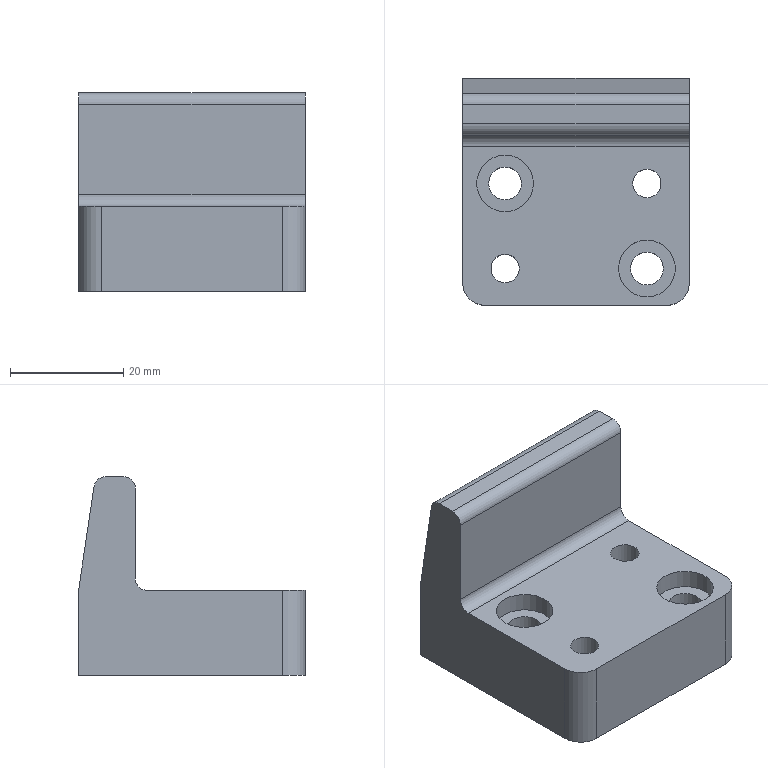Component | NX | GUIDE_BLOCK | 1 solid | 22 faces | volume 28956 mm3 | cylinder 11 | plane 11 | commonest cylinder face diameters 4 x3 5.8 x2 5 x2 8 x2 10 x2